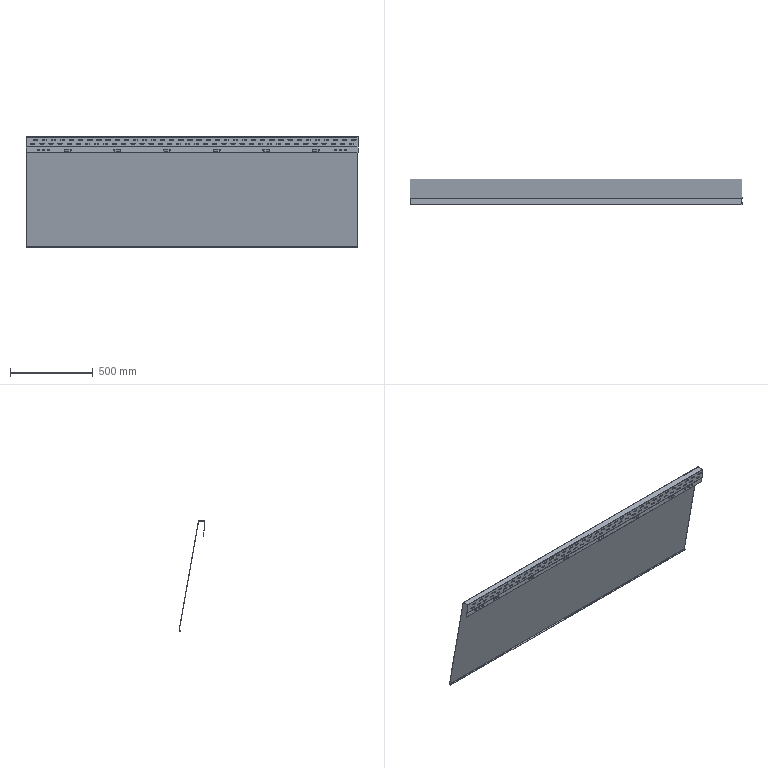Component | SolidWorks | Assembly2-1_TopCover2-1 | 1 solid | 406 faces | volume 2465609 mm3 | plane 204 | cylinder 202 | commonest cylinder face diameters 6 x144 11 x48 3.4 x5 0.4 x5